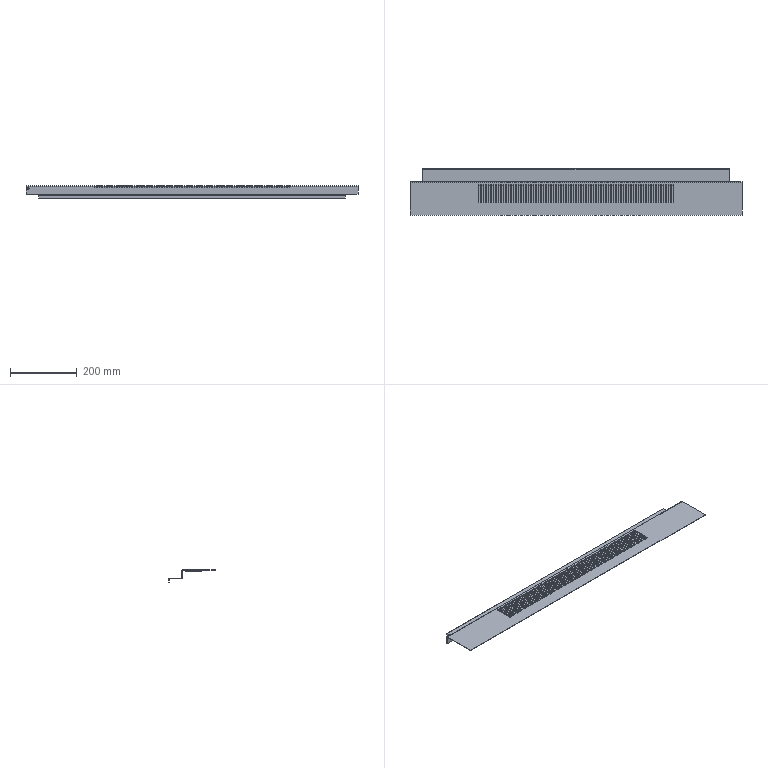Component | SolidWorks | AirFurnaceElectricalCabinet-FrontDoorLowerPlate-1 | 1 solid | 860 faces | volume 202583 mm3 | cylinder 480 | plane 380 | commonest cylinder face diameters 6 x236 8.4 x118 3.6 x118 1.5 x3 3.9 x3 6.5 x2